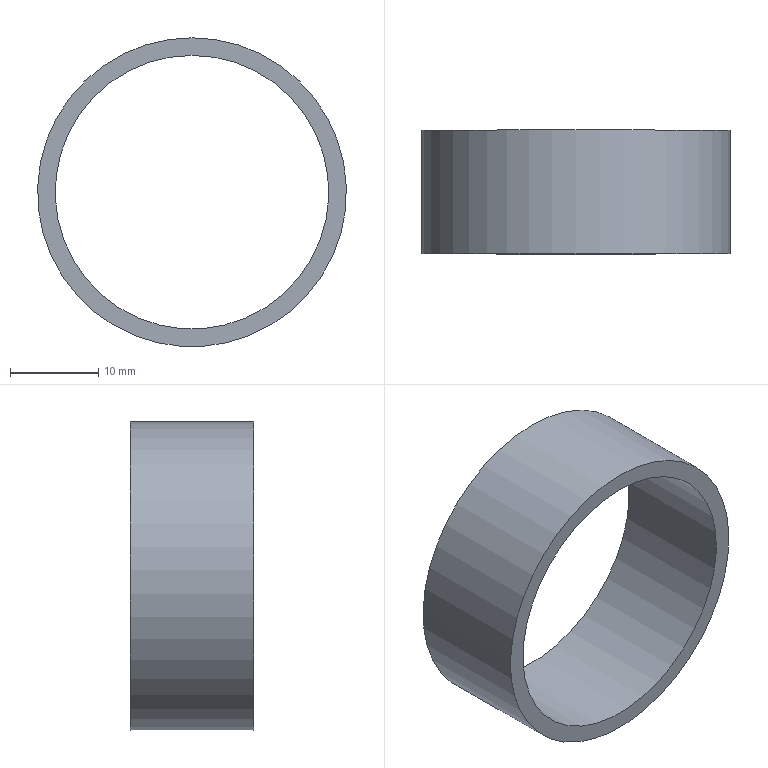Component | NX | BUSHING | 1 solid | 4 faces | box 35 x 14 x 35 mm | volume 2903 mm3 | cylinder 2 | plane 2 | commonest cylinder face diameters 35 x1 31 x1
STEP:
#1=CARTESIAN_POINT('',(0.,0.,0.));
#2=DIRECTION('',(0.,0.,1.));
#3=DIRECTION('',(1.,0.,0.));
#4=AXIS2_PLACEMENT_3D('',#1,#2,#3);
#5=CARTESIAN_POINT('',(630.189,-293.302,-1458.5));
#6=VERTEX_POINT('',#5);
#7=CARTESIAN_POINT('',(630.189,-293.302,-1476.));
#8=DIRECTION('',(0.,1.,0.));
#9=DIRECTION('',(0.,0.,1.));
#10=AXIS2_PLACEMENT_3D('',#7,#8,#9);
#11=CIRCLE('',#10,17.5);
#12=CARTESIAN_POINT('',(630.189,-293.302,-1476.));
#13=DIRECTION('',(0.,-1.,0.));
#14=DIRECTION('',(0.,0.,-1.));
#15=AXIS2_PLACEMENT_3D('',#12,#13,#14);
#16=CYLINDRICAL_SURFACE('',#15,17.5);
#17=CARTESIAN_POINT('',(9.425,0.));
#18=DIRECTION('',(-1.,0.));
#19=VECTOR('',#18,1.);
#20=LINE('',#17,#19);
#21=(GEOMETRIC_REPRESENTATION_CONTEXT(2)PARAMETRIC_REPRESENTATION_CONTEXT()REPRESENTATION_CONTEXT('',''));
#22=DEFINITIONAL_REPRESENTATION('',(#20),#21);
#23=PCURVE('',#16,#22);
#24=CARTESIAN_POINT('',(630.189,-293.302,-1476.));
#25=DIRECTION('',(0.,1.,0.));
#26=DIRECTION('',(0.,0.,1.));
#27=AXIS2_PLACEMENT_3D('',#24,#25,#26);
#28=PLANE('',#27);
#29=CARTESIAN_POINT('',(0.,0.));
#30=DIRECTION('',(1.,0.));
#31=AXIS2_PLACEMENT_2D('',#29,#30);
#32=CIRCLE('',#31,17.5);
#33=(GEOMETRIC_REPRESENTATION_CONTEXT(2)PARAMETRIC_REPRESENTATION_CONTEXT()REPRESENTATION_CONTEXT('',''));
#34=DEFINITIONAL_REPRESENTATION('',(#32),#33);
#35=PCURVE('',#28,#34);
#36=SURFACE_CURVE('',#11,(#23,#35),.PCURVE_S1.);
#37=EDGE_CURVE('',#6,#6,#36,.T.);
#38=ORIENTED_EDGE('',*,*,#37,.F.);
#39=CARTESIAN_POINT('',(630.189,-307.302,-1458.5));
#40=VERTEX_POINT('',#39);
#41=CARTESIAN_POINT('',(630.189,-293.302,-1458.5));
#42=CARTESIAN_POINT('',(630.189,-307.302,-1458.5));
#43=B_SPLINE_CURVE_WITH_KNOTS('',1,(#41,#42),.UNSPECIFIED.,.F.,.F.,(2,2),(0.,14.),.PIECEWISE_BEZIER_KNOTS.);
#44=CARTESIAN_POINT('',(9.425,0.));
#45=DIRECTION('',(0.,1.));
#46=VECTOR('',#45,1.);
#47=LINE('',#44,#46);
#48=(GEOMETRIC_REPRESENTATION_CONTEXT(2)PARAMETRIC_REPRESENTATION_CONTEXT()REPRESENTATION_CONTEXT('',''));
#49=DEFINITIONAL_REPRESENTATION('',(#47),#48);
#50=PCURVE('',#16,#49);
#51=CARTESIAN_POINT('',(3.142,0.));
#52=DIRECTION('',(0.,1.));
#53=VECTOR('',#52,1.);
#54=LINE('',#51,#53);
#55=(GEOMETRIC_REPRESENTATION_CONTEXT(2)PARAMETRIC_REPRESENTATION_CONTEXT()REPRESENTATION_CONTEXT('',''));
#56=DEFINITIONAL_REPRESENTATION('',(#54),#55);
#57=PCURVE('',#16,#56);
#58=SEAM_CURVE('',#43,(#50,#57),.PCURVE_S1.);
#59=EDGE_CURVE('',#6,#40,#58,.T.);
#60=ORIENTED_EDGE('',*,*,#59,.T.);
#61=CARTESIAN_POINT('',(630.189,-307.302,-1476.));
#62=DIRECTION('',(0.,1.,0.));
#63=DIRECTION('',(0.,0.,1.));
#64=AXIS2_PLACEMENT_3D('',#61,#62,#63);
#65=CIRCLE('',#64,17.5);
#66=CARTESIAN_POINT('',(9.425,14.));
#67=DIRECTION('',(-1.,0.));
#68=VECTOR('',#67,1.);
#69=LINE('',#66,#68);
#70=(GEOMETRIC_REPRESENTATION_CONTEXT(2)PARAMETRIC_REPRESENTATION_CONTEXT()REPRESENTATION_CONTEXT('',''));
#71=DEFINITIONAL_REPRESENTATION('',(#69),#70);
#72=PCURVE('',#16,#71);
#73=CARTESIAN_POINT('',(630.189,-307.302,-1476.));
#74=DIRECTION('',(0.,1.,0.));
#75=DIRECTION('',(0.,0.,1.));
#76=AXIS2_PLACEMENT_3D('',#73,#74,#75);
#77=PLANE('',#76);
#78=CARTESIAN_POINT('',(0.,0.));
#79=DIRECTION('',(1.,0.));
#80=AXIS2_PLACEMENT_2D('',#78,#79);
#81=CIRCLE('',#80,17.5);
#82=(GEOMETRIC_REPRESENTATION_CONTEXT(2)PARAMETRIC_REPRESENTATION_CONTEXT()REPRESENTATION_CONTEXT('',''));
#83=DEFINITIONAL_REPRESENTATION('',(#81),#82);
#84=PCURVE('',#77,#83);
#85=SURFACE_CURVE('',#65,(#72,#84),.PCURVE_S1.);
#86=EDGE_CURVE('',#40,#40,#85,.T.);
#87=ORIENTED_EDGE('',*,*,#86,.T.);
#88=ORIENTED_EDGE('',*,*,#59,.F.);
#89=EDGE_LOOP('',(#38,#60,#87,#88));
#90=FACE_BOUND('',#89,.T.);
#91=ADVANCED_FACE('',(#90),#16,.T.);
#92=CARTESIAN_POINT('',(630.189,-293.302,-1460.5));
#93=VERTEX_POINT('',#92);
#94=CARTESIAN_POINT('',(630.189,-293.302,-1476.));
#95=DIRECTION('',(0.,1.,0.));
#96=DIRECTION('',(0.,0.,1.));
#97=AXIS2_PLACEMENT_3D('',#94,#95,#96);
#98=CIRCLE('',#97,15.5);
#99=CARTESIAN_POINT('',(630.189,-293.302,-1476.));
#100=DIRECTION('',(0.,-1.,0.));
#101=DIRECTION('',(0.,0.,-1.));
#102=AXIS2_PLACEMENT_3D('',#99,#100,#101);
#103=CYLINDRICAL_SURFACE('',#102,15.5);
#104=CARTESIAN_POINT('',(9.425,0.));
#105=DIRECTION('',(-1.,0.));
#106=VECTOR('',#105,1.);
#107=LINE('',#104,#106);
#108=(GEOMETRIC_REPRESENTATION_CONTEXT(2)PARAMETRIC_REPRESENTATION_CONTEXT()REPRESENTATION_CONTEXT('',''));
#109=DEFINITIONAL_REPRESENTATION('',(#107),#108);
#110=PCURVE('',#103,#109);
#111=CARTESIAN_POINT('',(0.,0.));
#112=DIRECTION('',(1.,0.));
#113=AXIS2_PLACEMENT_2D('',#111,#112);
#114=CIRCLE('',#113,15.5);
#115=(GEOMETRIC_REPRESENTATION_CONTEXT(2)PARAMETRIC_REPRESENTATION_CONTEXT()REPRESENTATION_CONTEXT('',''));
#116=DEFINITIONAL_REPRESENTATION('',(#114),#115);
#117=PCURVE('',#28,#116);
#118=SURFACE_CURVE('',#98,(#110,#117),.PCURVE_S1.);
#119=EDGE_CURVE('',#93,#93,#118,.T.);
#120=ORIENTED_EDGE('',*,*,#119,.F.);
#121=CARTESIAN_POINT('',(630.189,-307.302,-1460.5));
#122=VERTEX_POINT('',#121);
#123=CARTESIAN_POINT('',(630.189,-293.302,-1460.5));
#124=CARTESIAN_POINT('',(630.189,-307.302,-1460.5));
#125=B_SPLINE_CURVE_WITH_KNOTS('',1,(#123,#124),.UNSPECIFIED.,.F.,.F.,(2,2),(0.,14.),.PIECEWISE_BEZIER_KNOTS.);
#126=CARTESIAN_POINT('',(9.425,0.));
#127=DIRECTION('',(0.,1.));
#128=VECTOR('',#127,1.);
#129=LINE('',#126,#128);
#130=(GEOMETRIC_REPRESENTATION_CONTEXT(2)PARAMETRIC_REPRESENTATION_CONTEXT()REPRESENTATION_CONTEXT('',''));
#131=DEFINITIONAL_REPRESENTATION('',(#129),#130);
#132=PCURVE('',#103,#131);
#133=CARTESIAN_POINT('',(3.142,0.));
#134=DIRECTION('',(0.,1.));
#135=VECTOR('',#134,1.);
#136=LINE('',#133,#135);
#137=(GEOMETRIC_REPRESENTATION_CONTEXT(2)PARAMETRIC_REPRESENTATION_CONTEXT()REPRESENTATION_CONTEXT('',''));
#138=DEFINITIONAL_REPRESENTATION('',(#136),#137);
#139=PCURVE('',#103,#138);
#140=SEAM_CURVE('',#125,(#132,#139),.PCURVE_S1.);
#141=EDGE_CURVE('',#93,#122,#140,.T.);
#142=ORIENTED_EDGE('',*,*,#141,.T.);
#143=CARTESIAN_POINT('',(630.189,-307.302,-1476.));
#144=DIRECTION('',(0.,1.,0.));
#145=DIRECTION('',(0.,0.,1.));
#146=AXIS2_PLACEMENT_3D('',#143,#144,#145);
#147=CIRCLE('',#146,15.5);
#148=CARTESIAN_POINT('',(9.425,14.));
#149=DIRECTION('',(-1.,0.));
#150=VECTOR('',#149,1.);
#151=LINE('',#148,#150);
#152=(GEOMETRIC_REPRESENTATION_CONTEXT(2)PARAMETRIC_REPRESENTATION_CONTEXT()REPRESENTATION_CONTEXT('',''));
#153=DEFINITIONAL_REPRESENTATION('',(#151),#152);
#154=PCURVE('',#103,#153);
#155=CARTESIAN_POINT('',(0.,0.));
#156=DIRECTION('',(1.,0.));
#157=AXIS2_PLACEMENT_2D('',#155,#156);
#158=CIRCLE('',#157,15.5);
#159=(GEOMETRIC_REPRESENTATION_CONTEXT(2)PARAMETRIC_REPRESENTATION_CONTEXT()REPRESENTATION_CONTEXT('',''));
#160=DEFINITIONAL_REPRESENTATION('',(#158),#159);
#161=PCURVE('',#77,#160);
#162=SURFACE_CURVE('',#147,(#154,#161),.PCURVE_S1.);
#163=EDGE_CURVE('',#122,#122,#162,.T.);
#164=ORIENTED_EDGE('',*,*,#163,.T.);
#165=ORIENTED_EDGE('',*,*,#141,.F.);
#166=EDGE_LOOP('',(#120,#142,#164,#165));
#167=FACE_BOUND('',#166,.F.);
#168=ADVANCED_FACE('',(#167),#103,.F.);
#169=ORIENTED_EDGE('',*,*,#37,.T.);
#170=EDGE_LOOP('',(#169));
#171=FACE_BOUND('',#170,.T.);
#172=ORIENTED_EDGE('',*,*,#119,.F.);
#173=EDGE_LOOP('',(#172));
#174=FACE_BOUND('',#173,.T.);
#175=ADVANCED_FACE('',(#171,#174),#28,.T.);
#176=ORIENTED_EDGE('',*,*,#86,.F.);
#177=EDGE_LOOP('',(#176));
#178=FACE_BOUND('',#177,.T.);
#179=ORIENTED_EDGE('',*,*,#163,.T.);
#180=EDGE_LOOP('',(#179));
#181=FACE_BOUND('',#180,.T.);
#182=ADVANCED_FACE('',(#178,#181),#77,.F.);
#183=CLOSED_SHELL('',(#91,#168,#175,#182));
#184=MANIFOLD_SOLID_BREP('',#183);
#185=(LENGTH_UNIT()NAMED_UNIT(*)SI_UNIT(.MILLI.,.METRE.));
#186=UNCERTAINTY_MEASURE_WITH_UNIT(LENGTH_MEASURE(0.00001),#185,'','');
#187=(NAMED_UNIT(*)PLANE_ANGLE_UNIT()SI_UNIT($,.RADIAN.));
#188=(NAMED_UNIT(*)SI_UNIT($,.STERADIAN.)SOLID_ANGLE_UNIT());
#189=(GEOMETRIC_REPRESENTATION_CONTEXT(3)GLOBAL_UNCERTAINTY_ASSIGNED_CONTEXT((#186))GLOBAL_UNIT_ASSIGNED_CONTEXT((#185,#187,#188))REPRESENTATION_CONTEXT('',''));
#190=ADVANCED_BREP_SHAPE_REPRESENTATION('',(#4,#184),#189);